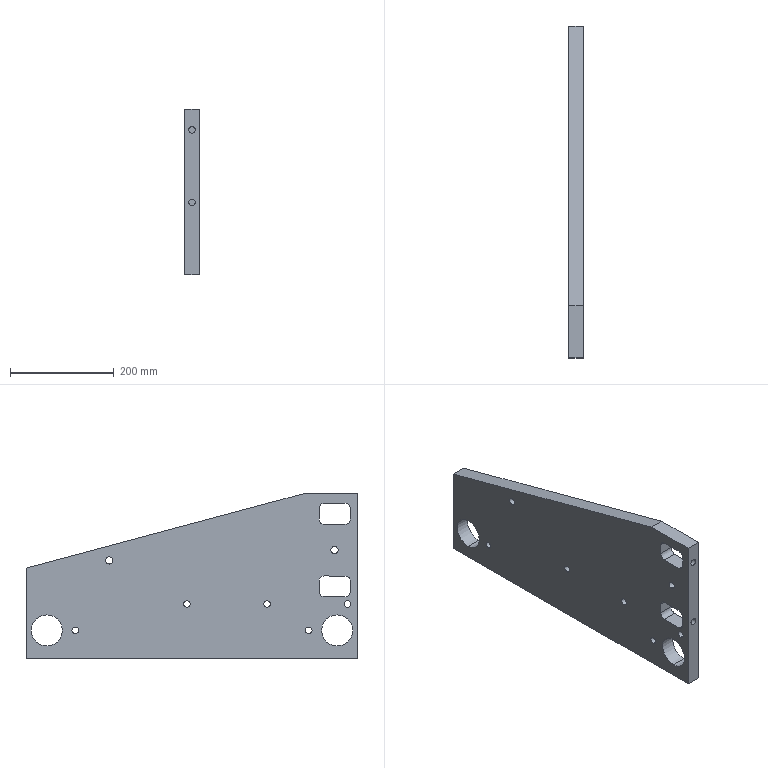Component | SolidWorks | Assembly2-1_MainBracket-2 | 1 solid | 45 faces | box 28 x 640 x 320 mm | volume 4321410 mm3 | cylinder 30 | plane 15 | commonest cylinder face diameters 13 x14 20 x8 14 x4 60 x4
build123d program:
from build123d import *

# Parameters (mm, degrees)
SKETCH1_W           = 110
SKETCH1_H           = 640
SKETCH1_R           = 30
BOSS_EXTRUDE1_DEPTH = 28
SKETCH4_R           = 6.5
CUT_EXTRUDE1_DEPTH  = 326.897
BOSS_EXTRUDE2_DEPTH = 28
CUT_EXTRUDE2_DEPTH  = 417.424
SKETCH8_R           = 6.5
CUT_EXTRUDE3_DEPTH  = 20
SKETCH9_R           = 7
CUT_EXTRUDE4_DEPTH  = 417.424
SKETCH10_R          = 7
CUT_EXTRUDE5_DEPTH  = 417.424
SKETCH11_R          = 6.5
CUT_EXTRUDE6_DEPTH  = 417.424


with BuildPart() as part:
    # Sketch1 → Boss-Extrude1 (new body)
    with BuildSketch(Plane.XY):
        Rectangle(SKETCH1_W, SKETCH1_H)
        with Locations((0, 280)):
            Circle(SKETCH1_R, mode=Mode.SUBTRACT)
        with Locations(Location((0, -280, 0), (0, 0, 180))):
            Circle(SKETCH1_R, mode=Mode.SUBTRACT)
    extrude(amount=BOSS_EXTRUDE1_DEPTH)

    # Sketch4 → Cut-Extrude1 (cut, through all)
    with BuildSketch(Plane.XY.offset(28)):
        with Locations((0, 225)):
            Circle(SKETCH4_R)
        with Locations(Location((0, -225, 0), (0, 0, 180))):
            Circle(SKETCH4_R)
    extrude(amount=-CUT_EXTRUDE1_DEPTH, mode=Mode.SUBTRACT)

    # Sketch6 → Boss-Extrude2 (add, through all)
    with BuildSketch(Plane.XY.offset(28)):
        Polygon((265, -220), (120.307, 320), (55, 320), (55, -320), (265, -320), align=None)
    extrude(amount=-BOSS_EXTRUDE2_DEPTH)

    # Sketch7 → Cut-Extrude2 (cut, through all)
    with BuildSketch(Plane.XY.offset(28)):
        with BuildLine():
            Line((235, -305), (215, -305))
            ThreePointArc((215, -305), (207.929, -302.071), (205, -295))
            Line((205, -295), (205, -255))
            ThreePointArc((205, -255), (207.929, -247.929), (215, -245))
            Line((215, -245), (235, -245))
            ThreePointArc((235, -245), (242.071, -247.929), (245, -255))
            Line((245, -255), (245, -295))
            ThreePointArc((245, -295), (242.071, -302.071), (235, -305))
        make_face()
        with BuildLine():
            Line((105, -295), (105, -255))
            ThreePointArc((105, -255), (102.071, -247.929), (95, -245))
            Line((95, -245), (75, -245))
            ThreePointArc((75, -245), (67.929, -247.929), (65, -255))
            Line((65, -255), (65, -295))
            ThreePointArc((65, -295), (67.929, -302.071), (75, -305))
            Line((75, -305), (95, -305))
            ThreePointArc((95, -305), (102.071, -302.071), (105, -295))
        make_face()
    extrude(amount=-CUT_EXTRUDE2_DEPTH, mode=Mode.SUBTRACT)

    # Sketch8 → Cut-Extrude3 (cut)
    with BuildSketch(Plane.XZ.offset(320)):
        with Locations(Location((85, 14, 0), (0, 0, 270))):
            Circle(SKETCH8_R)
        with Locations(Location((225, 14, 0), (0, 0, 270))):
            Circle(SKETCH8_R)
    extrude(amount=-CUT_EXTRUDE3_DEPTH, mode=Mode.SUBTRACT)

    # Sketch9 → Cut-Extrude4 (cut, through all)
    with BuildSketch(Plane.XY.offset(28)):
        with Locations((155, -275)):
            Circle(SKETCH9_R)
    extrude(amount=-CUT_EXTRUDE4_DEPTH, mode=Mode.SUBTRACT)

    # Sketch10 → Cut-Extrude5 (cut, through all)
    with BuildSketch(Plane.XY.offset(28)):
        with Locations((135, 160)):
            Circle(SKETCH10_R)
    extrude(amount=-CUT_EXTRUDE5_DEPTH, mode=Mode.SUBTRACT)

    # Sketch11 → Cut-Extrude6 (cut, through all)
    with BuildSketch(Plane.XY.offset(28)):
        with Locations((51, 10)):
            Circle(SKETCH11_R)
        with Locations((51, -145)):
            Circle(SKETCH11_R)
        with Locations((51, -300)):
            Circle(SKETCH11_R)
    extrude(amount=-CUT_EXTRUDE6_DEPTH, mode=Mode.SUBTRACT)


solid = part.part

# Placed as in the assembly
solid = solid.moved(Location((346.98, -4.181, 0), (0, -90, 0)))